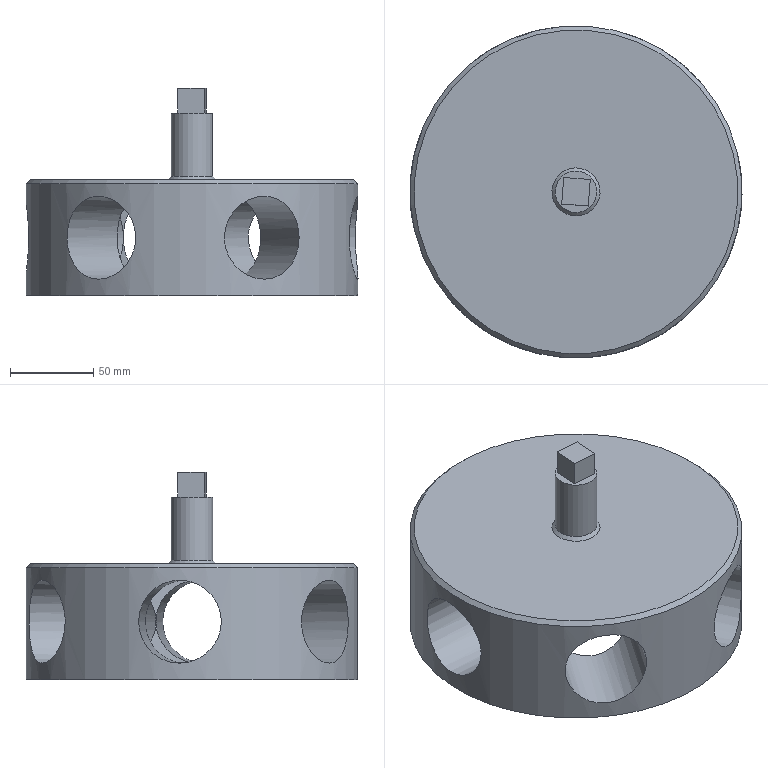Component | NX | ROTOR | 1 solid | 26 faces | volume 1150770 mm3 | cylinder 15 | plane 9 | cone 2 | commonest cylinder face diameters 100 x7 50 x6 200 x1 25 x1